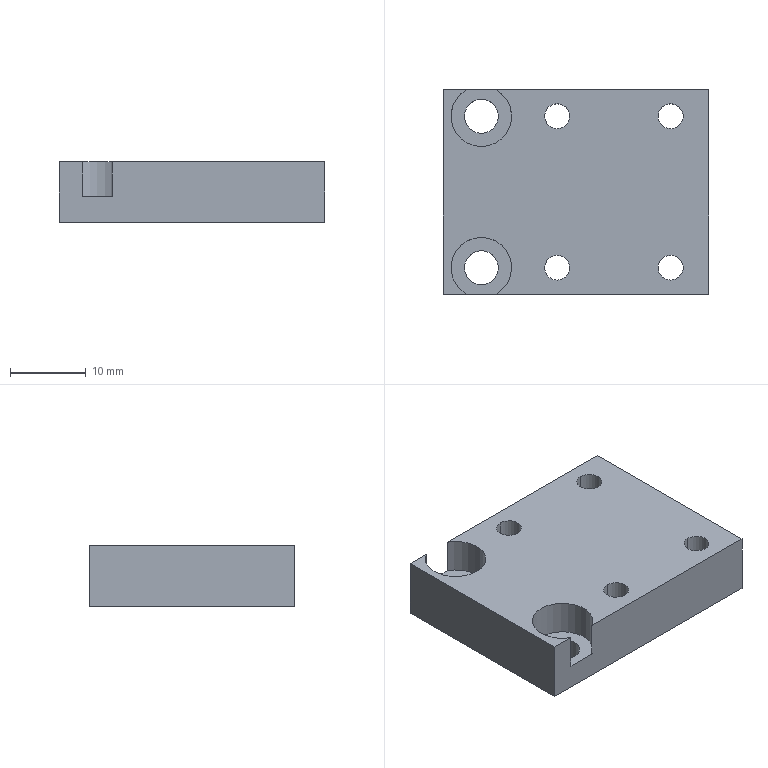Component | SolidWorks | JQ-2-0-005-1 | 1 solid | 23 faces | box 35 x 27 x 8 mm | volume 6728 mm3 | cylinder 15 | plane 8 | commonest cylinder face diameters 3.3 x8 4.5 x4 8 x3
build123d program:
from build123d import *

# Parameters (mm, degrees)
SKETCH1_W                                            = 27
SKETCH1_H                                            = 35
BOSS_EXTRUDE1_DEPTH                                  = 8
HOLE_SIZE_ACCORDING_TO_TYPE_1_OF_HEX_SOC_D           = 4.5
HOLE_SIZE_ACCORDING_TO_TYPE_1_OF_HEX_SOC_CBORE_D     = 8
HOLE_SIZE_ACCORDING_TO_TYPE_1_OF_HEX_SOC_CBORE_DEPTH = 4.6
M4_TAPPED_HOLE1_D                                    = 3.3
M4_TAPPED_HOLE1_DEPTH                                = 11.5
M4_TAPPED_HOLE1_TIP                                  = 0.9914


with BuildPart() as part:
    # Sketch1 → Boss-Extrude1 (new body)
    with BuildSketch(Plane.XY):
        with Locations((13.5, 17.5)):
            Rectangle(SKETCH1_W, SKETCH1_H)
    extrude(amount=BOSS_EXTRUDE1_DEPTH)

    # Hole Size according to type 1 of hex soc (through all)
    with Locations(Plane.XY.offset(8)):
        with Locations((23.5, 5), (3.5, 5)):
            CounterBoreHole(HOLE_SIZE_ACCORDING_TO_TYPE_1_OF_HEX_SOC_D / 2, HOLE_SIZE_ACCORDING_TO_TYPE_1_OF_HEX_SOC_CBORE_D / 2, HOLE_SIZE_ACCORDING_TO_TYPE_1_OF_HEX_SOC_CBORE_DEPTH)

    # M4 Tapped Hole1
    with Locations(Plane.XY.offset(8)):
        with Locations((23.5, 30), (3.5, 30), (3.5, 15), (23.5, 15)):
            Hole(M4_TAPPED_HOLE1_D / 2, depth=M4_TAPPED_HOLE1_DEPTH)
            with Locations((0, 0, -(M4_TAPPED_HOLE1_DEPTH + M4_TAPPED_HOLE1_TIP / 2))):  # 118° drill point
                Cone(0, M4_TAPPED_HOLE1_D / 2, M4_TAPPED_HOLE1_TIP, mode=Mode.SUBTRACT)


solid = part.part

# Placed as in the assembly
solid = solid.moved(Location((-170.058, 42.839, 99.131), (0, 0, -90)))
STEP:
#1=CARTESIAN_POINT('',(-5.514,0.6964,3.903));
#2=VERTEX_POINT('',#1);
#3=CARTESIAN_POINT('',(-5.514,0.8263,3.903));
#4=VERTEX_POINT('',#3);
#5=CARTESIAN_POINT('',(-5.514,0.7614,3.903));
#6=DIRECTION('',(-0.,-0.,-1.));
#7=DIRECTION('',(0.,1.,0.));
#8=AXIS2_PLACEMENT_3D('',#5,#6,#7);
#9=CIRCLE('',#8,0.06496);
#10=EDGE_CURVE('',#2,#4,#9,.T.);
#11=ORIENTED_EDGE('',*,*,#10,.T.);
#12=CARTESIAN_POINT('',(-5.514,0.8263,4.218));
#13=VERTEX_POINT('',#12);
#14=CARTESIAN_POINT('',(-5.514,0.8263,4.218));
#15=DIRECTION('',(0.,0.,1.));
#16=VECTOR('',#15,39.37);
#17=LINE('',#14,#16);
#18=EDGE_CURVE('',#4,#13,#17,.T.);
#19=ORIENTED_EDGE('',*,*,#18,.T.);
#20=CARTESIAN_POINT('',(-5.514,0.6964,4.218));
#21=VERTEX_POINT('',#20);
#22=CARTESIAN_POINT('',(-5.514,0.7614,4.218));
#23=DIRECTION('',(0.,0.,1.));
#24=DIRECTION('',(0.,-1.,0.));
#25=AXIS2_PLACEMENT_3D('',#22,#23,#24);
#26=CIRCLE('',#25,0.06496);
#27=EDGE_CURVE('',#13,#21,#26,.T.);
#28=ORIENTED_EDGE('',*,*,#27,.T.);
#29=CARTESIAN_POINT('',(-5.514,0.6964,4.218));
#30=DIRECTION('',(0.,0.,1.));
#31=VECTOR('',#30,39.37);
#32=LINE('',#29,#31);
#33=EDGE_CURVE('',#2,#21,#32,.T.);
#34=ORIENTED_EDGE('',*,*,#33,.F.);
#35=EDGE_LOOP('',(#11,#19,#28,#34));
#36=FACE_OUTER_BOUND('',#35,.T.);
#37=CARTESIAN_POINT('',(-5.514,0.7614,4.218));
#38=DIRECTION('',(0.,0.,1.));
#39=DIRECTION('',(0.,-1.,0.));
#40=AXIS2_PLACEMENT_3D('',#37,#38,#39);
#41=CYLINDRICAL_SURFACE('',#40,0.06496);
#42=ADVANCED_FACE('',(#36),#41,.F.);
#43=CARTESIAN_POINT('',(-5.514,1.484,3.903));
#44=VERTEX_POINT('',#43);
#45=CARTESIAN_POINT('',(-5.514,1.614,3.903));
#46=VERTEX_POINT('',#45);
#47=CARTESIAN_POINT('',(-5.514,1.549,3.903));
#48=DIRECTION('',(-0.,-0.,-1.));
#49=DIRECTION('',(0.,1.,0.));
#50=AXIS2_PLACEMENT_3D('',#47,#48,#49);
#51=CIRCLE('',#50,0.06496);
#52=EDGE_CURVE('',#44,#46,#51,.T.);
#53=ORIENTED_EDGE('',*,*,#52,.T.);
#54=CARTESIAN_POINT('',(-5.514,1.614,4.218));
#55=VERTEX_POINT('',#54);
#56=CARTESIAN_POINT('',(-5.514,1.614,4.218));
#57=DIRECTION('',(0.,0.,1.));
#58=VECTOR('',#57,39.37);
#59=LINE('',#56,#58);
#60=EDGE_CURVE('',#46,#55,#59,.T.);
#61=ORIENTED_EDGE('',*,*,#60,.T.);
#62=CARTESIAN_POINT('',(-5.514,1.484,4.218));
#63=VERTEX_POINT('',#62);
#64=CARTESIAN_POINT('',(-5.514,1.549,4.218));
#65=DIRECTION('',(0.,0.,1.));
#66=DIRECTION('',(0.,-1.,0.));
#67=AXIS2_PLACEMENT_3D('',#64,#65,#66);
#68=CIRCLE('',#67,0.06496);
#69=EDGE_CURVE('',#55,#63,#68,.T.);
#70=ORIENTED_EDGE('',*,*,#69,.T.);
#71=CARTESIAN_POINT('',(-5.514,1.484,4.218));
#72=DIRECTION('',(0.,0.,1.));
#73=VECTOR('',#72,39.37);
#74=LINE('',#71,#73);
#75=EDGE_CURVE('',#44,#63,#74,.T.);
#76=ORIENTED_EDGE('',*,*,#75,.F.);
#77=EDGE_LOOP('',(#53,#61,#70,#76));
#78=FACE_OUTER_BOUND('',#77,.T.);
#79=CARTESIAN_POINT('',(-5.514,1.549,4.218));
#80=DIRECTION('',(0.,0.,1.));
#81=DIRECTION('',(0.,-1.,0.));
#82=AXIS2_PLACEMENT_3D('',#79,#80,#81);
#83=CYLINDRICAL_SURFACE('',#82,0.06496);
#84=ADVANCED_FACE('',(#78),#83,.F.);
#85=CARTESIAN_POINT('',(-6.105,1.484,3.903));
#86=VERTEX_POINT('',#85);
#87=CARTESIAN_POINT('',(-6.105,1.614,3.903));
#88=VERTEX_POINT('',#87);
#89=CARTESIAN_POINT('',(-6.105,1.549,3.903));
#90=DIRECTION('',(-0.,-0.,-1.));
#91=DIRECTION('',(0.,1.,0.));
#92=AXIS2_PLACEMENT_3D('',#89,#90,#91);
#93=CIRCLE('',#92,0.06496);
#94=EDGE_CURVE('',#86,#88,#93,.T.);
#95=ORIENTED_EDGE('',*,*,#94,.T.);
#96=CARTESIAN_POINT('',(-6.105,1.614,4.218));
#97=VERTEX_POINT('',#96);
#98=CARTESIAN_POINT('',(-6.105,1.614,4.218));
#99=DIRECTION('',(0.,0.,1.));
#100=VECTOR('',#99,39.37);
#101=LINE('',#98,#100);
#102=EDGE_CURVE('',#88,#97,#101,.T.);
#103=ORIENTED_EDGE('',*,*,#102,.T.);
#104=CARTESIAN_POINT('',(-6.105,1.484,4.218));
#105=VERTEX_POINT('',#104);
#106=CARTESIAN_POINT('',(-6.105,1.549,4.218));
#107=DIRECTION('',(0.,0.,1.));
#108=DIRECTION('',(0.,-1.,0.));
#109=AXIS2_PLACEMENT_3D('',#106,#107,#108);
#110=CIRCLE('',#109,0.06496);
#111=EDGE_CURVE('',#97,#105,#110,.T.);
#112=ORIENTED_EDGE('',*,*,#111,.T.);
#113=CARTESIAN_POINT('',(-6.105,1.484,4.218));
#114=DIRECTION('',(0.,0.,1.));
#115=VECTOR('',#114,39.37);
#116=LINE('',#113,#115);
#117=EDGE_CURVE('',#86,#105,#116,.T.);
#118=ORIENTED_EDGE('',*,*,#117,.F.);
#119=EDGE_LOOP('',(#95,#103,#112,#118));
#120=FACE_OUTER_BOUND('',#119,.T.);
#121=CARTESIAN_POINT('',(-6.105,1.549,4.218));
#122=DIRECTION('',(0.,0.,1.));
#123=DIRECTION('',(0.,-1.,0.));
#124=AXIS2_PLACEMENT_3D('',#121,#122,#123);
#125=CYLINDRICAL_SURFACE('',#124,0.06496);
#126=ADVANCED_FACE('',(#120),#125,.F.);
#127=CARTESIAN_POINT('',(-6.105,0.6964,3.903));
#128=VERTEX_POINT('',#127);
#129=CARTESIAN_POINT('',(-6.105,0.8263,3.903));
#130=VERTEX_POINT('',#129);
#131=CARTESIAN_POINT('',(-6.105,0.7614,3.903));
#132=DIRECTION('',(-0.,-0.,-1.));
#133=DIRECTION('',(0.,1.,0.));
#134=AXIS2_PLACEMENT_3D('',#131,#132,#133);
#135=CIRCLE('',#134,0.06496);
#136=EDGE_CURVE('',#128,#130,#135,.T.);
#137=ORIENTED_EDGE('',*,*,#136,.T.);
#138=CARTESIAN_POINT('',(-6.105,0.8263,4.218));
#139=VERTEX_POINT('',#138);
#140=CARTESIAN_POINT('',(-6.105,0.8263,4.218));
#141=DIRECTION('',(0.,0.,1.));
#142=VECTOR('',#141,39.37);
#143=LINE('',#140,#142);
#144=EDGE_CURVE('',#130,#139,#143,.T.);
#145=ORIENTED_EDGE('',*,*,#144,.T.);
#146=CARTESIAN_POINT('',(-6.105,0.6964,4.218));
#147=VERTEX_POINT('',#146);
#148=CARTESIAN_POINT('',(-6.105,0.7614,4.218));
#149=DIRECTION('',(0.,0.,1.));
#150=DIRECTION('',(0.,-1.,0.));
#151=AXIS2_PLACEMENT_3D('',#148,#149,#150);
#152=CIRCLE('',#151,0.06496);
#153=EDGE_CURVE('',#139,#147,#152,.T.);
#154=ORIENTED_EDGE('',*,*,#153,.T.);
#155=CARTESIAN_POINT('',(-6.105,0.6964,4.218));
#156=DIRECTION('',(0.,0.,1.));
#157=VECTOR('',#156,39.37);
#158=LINE('',#155,#157);
#159=EDGE_CURVE('',#128,#147,#158,.T.);
#160=ORIENTED_EDGE('',*,*,#159,.F.);
#161=EDGE_LOOP('',(#137,#145,#154,#160));
#162=FACE_OUTER_BOUND('',#161,.T.);
#163=CARTESIAN_POINT('',(-6.105,0.7614,4.218));
#164=DIRECTION('',(0.,0.,1.));
#165=DIRECTION('',(0.,-1.,0.));
#166=AXIS2_PLACEMENT_3D('',#163,#164,#165);
#167=CYLINDRICAL_SURFACE('',#166,0.06496);
#168=ADVANCED_FACE('',(#162),#167,.F.);
#169=CARTESIAN_POINT('',(-6.498,0.85,3.903));
#170=VERTEX_POINT('',#169);
#171=CARTESIAN_POINT('',(-6.498,0.6728,3.903));
#172=VERTEX_POINT('',#171);
#173=CARTESIAN_POINT('',(-6.498,0.7614,3.903));
#174=DIRECTION('',(0.,0.,1.));
#175=DIRECTION('',(0.,-1.,0.));
#176=AXIS2_PLACEMENT_3D('',#173,#174,#175);
#177=CIRCLE('',#176,0.08858);
#178=EDGE_CURVE('',#170,#172,#177,.T.);
#179=ORIENTED_EDGE('',*,*,#178,.F.);
#180=CARTESIAN_POINT('',(-6.498,0.85,4.037));
#181=VERTEX_POINT('',#180);
#182=CARTESIAN_POINT('',(-6.498,0.85,4.218));
#183=DIRECTION('',(0.,0.,1.));
#184=VECTOR('',#183,39.37);
#185=LINE('',#182,#184);
#186=EDGE_CURVE('',#170,#181,#185,.T.);
#187=ORIENTED_EDGE('',*,*,#186,.T.);
#188=CARTESIAN_POINT('',(-6.498,0.6728,4.037));
#189=VERTEX_POINT('',#188);
#190=CARTESIAN_POINT('',(-6.498,0.7614,4.037));
#191=DIRECTION('',(0.,0.,1.));
#192=DIRECTION('',(0.,-1.,0.));
#193=AXIS2_PLACEMENT_3D('',#190,#191,#192);
#194=CIRCLE('',#193,0.08858);
#195=EDGE_CURVE('',#181,#189,#194,.T.);
#196=ORIENTED_EDGE('',*,*,#195,.T.);
#197=CARTESIAN_POINT('',(-6.498,0.6728,4.218));
#198=DIRECTION('',(0.,0.,1.));
#199=VECTOR('',#198,39.37);
#200=LINE('',#197,#199);
#201=EDGE_CURVE('',#172,#189,#200,.T.);
#202=ORIENTED_EDGE('',*,*,#201,.F.);
#203=EDGE_LOOP('',(#179,#187,#196,#202));
#204=FACE_OUTER_BOUND('',#203,.T.);
#205=CARTESIAN_POINT('',(-6.498,0.7614,4.218));
#206=DIRECTION('',(0.,0.,1.));
#207=DIRECTION('',(0.,-1.,0.));
#208=AXIS2_PLACEMENT_3D('',#205,#206,#207);
#209=CYLINDRICAL_SURFACE('',#208,0.08858);
#210=ADVANCED_FACE('',(#204),#209,.F.);
#211=CARTESIAN_POINT('',(-6.498,1.637,3.903));
#212=VERTEX_POINT('',#211);
#213=CARTESIAN_POINT('',(-6.498,1.46,3.903));
#214=VERTEX_POINT('',#213);
#215=CARTESIAN_POINT('',(-6.498,1.549,3.903));
#216=DIRECTION('',(0.,0.,1.));
#217=DIRECTION('',(0.,-1.,0.));
#218=AXIS2_PLACEMENT_3D('',#215,#216,#217);
#219=CIRCLE('',#218,0.08858);
#220=EDGE_CURVE('',#212,#214,#219,.T.);
#221=ORIENTED_EDGE('',*,*,#220,.F.);
#222=CARTESIAN_POINT('',(-6.498,1.637,4.037));
#223=VERTEX_POINT('',#222);
#224=CARTESIAN_POINT('',(-6.498,1.637,4.218));
#225=DIRECTION('',(0.,0.,1.));
#226=VECTOR('',#225,39.37);
#227=LINE('',#224,#226);
#228=EDGE_CURVE('',#212,#223,#227,.T.);
#229=ORIENTED_EDGE('',*,*,#228,.T.);
#230=CARTESIAN_POINT('',(-6.498,1.46,4.037));
#231=VERTEX_POINT('',#230);
#232=CARTESIAN_POINT('',(-6.498,1.549,4.037));
#233=DIRECTION('',(0.,0.,1.));
#234=DIRECTION('',(0.,-1.,0.));
#235=AXIS2_PLACEMENT_3D('',#232,#233,#234);
#236=CIRCLE('',#235,0.08858);
#237=EDGE_CURVE('',#223,#231,#236,.T.);
#238=ORIENTED_EDGE('',*,*,#237,.T.);
#239=CARTESIAN_POINT('',(-6.498,1.46,4.218));
#240=DIRECTION('',(0.,0.,1.));
#241=VECTOR('',#240,39.37);
#242=LINE('',#239,#241);
#243=EDGE_CURVE('',#214,#231,#242,.T.);
#244=ORIENTED_EDGE('',*,*,#243,.F.);
#245=EDGE_LOOP('',(#221,#229,#238,#244));
#246=FACE_OUTER_BOUND('',#245,.T.);
#247=CARTESIAN_POINT('',(-6.498,1.549,4.218));
#248=DIRECTION('',(0.,0.,1.));
#249=DIRECTION('',(0.,-1.,0.));
#250=AXIS2_PLACEMENT_3D('',#247,#248,#249);
#251=CYLINDRICAL_SURFACE('',#250,0.08858);
#252=ADVANCED_FACE('',(#246),#251,.F.);
#253=CARTESIAN_POINT('',(-6.498,1.391,4.037));
#254=VERTEX_POINT('',#253);
#255=CARTESIAN_POINT('',(-6.422,1.687,4.037));
#256=VERTEX_POINT('',#255);
#257=CARTESIAN_POINT('',(-6.498,1.549,4.037));
#258=DIRECTION('',(0.,0.,1.));
#259=DIRECTION('',(0.,-1.,0.));
#260=AXIS2_PLACEMENT_3D('',#257,#258,#259);
#261=CIRCLE('',#260,0.1575);
#262=EDGE_CURVE('',#254,#256,#261,.T.);
#263=ORIENTED_EDGE('',*,*,#262,.F.);
#264=CARTESIAN_POINT('',(-6.498,1.391,4.218));
#265=VERTEX_POINT('',#264);
#266=CARTESIAN_POINT('',(-6.498,1.391,4.218));
#267=DIRECTION('',(0.,0.,1.));
#268=VECTOR('',#267,39.37);
#269=LINE('',#266,#268);
#270=EDGE_CURVE('',#254,#265,#269,.T.);
#271=ORIENTED_EDGE('',*,*,#270,.T.);
#272=CARTESIAN_POINT('',(-6.422,1.687,4.218));
#273=VERTEX_POINT('',#272);
#274=CARTESIAN_POINT('',(-6.498,1.549,4.218));
#275=DIRECTION('',(-0.,-0.,-1.));
#276=DIRECTION('',(0.,1.,0.));
#277=AXIS2_PLACEMENT_3D('',#274,#275,#276);
#278=CIRCLE('',#277,0.1575);
#279=EDGE_CURVE('',#273,#265,#278,.T.);
#280=ORIENTED_EDGE('',*,*,#279,.F.);
#281=CARTESIAN_POINT('',(-6.422,1.687,4.218));
#282=DIRECTION('',(0.,0.,1.));
#283=VECTOR('',#282,39.37);
#284=LINE('',#281,#283);
#285=EDGE_CURVE('',#256,#273,#284,.T.);
#286=ORIENTED_EDGE('',*,*,#285,.F.);
#287=EDGE_LOOP('',(#263,#271,#280,#286));
#288=FACE_OUTER_BOUND('',#287,.T.);
#289=CARTESIAN_POINT('',(-6.498,1.549,4.218));
#290=DIRECTION('',(0.,0.,1.));
#291=DIRECTION('',(0.,-1.,0.));
#292=AXIS2_PLACEMENT_3D('',#289,#290,#291);
#293=CYLINDRICAL_SURFACE('',#292,0.1575);
#294=ADVANCED_FACE('',(#288),#293,.F.);
#295=CARTESIAN_POINT('',(-6.575,1.687,4.037));
#296=VERTEX_POINT('',#295);
#297=CARTESIAN_POINT('',(-6.695,1.687,4.037));
#298=DIRECTION('',(1.,-0.,-0.));
#299=VECTOR('',#298,39.37);
#300=LINE('',#297,#299);
#301=EDGE_CURVE('',#296,#256,#300,.T.);
#302=ORIENTED_EDGE('',*,*,#301,.T.);
#303=ORIENTED_EDGE('',*,*,#285,.T.);
#304=CARTESIAN_POINT('',(-5.317,1.687,4.218));
#305=VERTEX_POINT('',#304);
#306=CARTESIAN_POINT('',(-6.695,1.687,4.218));
#307=DIRECTION('',(-1.,0.,0.));
#308=VECTOR('',#307,39.37);
#309=LINE('',#306,#308);
#310=EDGE_CURVE('',#305,#273,#309,.T.);
#311=ORIENTED_EDGE('',*,*,#310,.F.);
#312=CARTESIAN_POINT('',(-5.317,1.687,3.903));
#313=VERTEX_POINT('',#312);
#314=CARTESIAN_POINT('',(-5.317,1.687,4.218));
#315=DIRECTION('',(-0.,-0.,-1.));
#316=VECTOR('',#315,39.37);
#317=LINE('',#314,#316);
#318=EDGE_CURVE('',#305,#313,#317,.T.);
#319=ORIENTED_EDGE('',*,*,#318,.T.);
#320=CARTESIAN_POINT('',(-6.695,1.687,3.903));
#321=VERTEX_POINT('',#320);
#322=CARTESIAN_POINT('',(-6.695,1.687,3.903));
#323=DIRECTION('',(-1.,0.,0.));
#324=VECTOR('',#323,39.37);
#325=LINE('',#322,#324);
#326=EDGE_CURVE('',#313,#321,#325,.T.);
#327=ORIENTED_EDGE('',*,*,#326,.T.);
#328=CARTESIAN_POINT('',(-6.695,1.687,4.218));
#329=VERTEX_POINT('',#328);
#330=CARTESIAN_POINT('',(-6.695,1.687,4.218));
#331=DIRECTION('',(-0.,-0.,-1.));
#332=VECTOR('',#331,39.37);
#333=LINE('',#330,#332);
#334=EDGE_CURVE('',#329,#321,#333,.T.);
#335=ORIENTED_EDGE('',*,*,#334,.F.);
#336=CARTESIAN_POINT('',(-6.575,1.687,4.218));
#337=VERTEX_POINT('',#336);
#338=CARTESIAN_POINT('',(-6.695,1.687,4.218));
#339=DIRECTION('',(-1.,0.,0.));
#340=VECTOR('',#339,39.37);
#341=LINE('',#338,#340);
#342=EDGE_CURVE('',#337,#329,#341,.T.);
#343=ORIENTED_EDGE('',*,*,#342,.F.);
#344=CARTESIAN_POINT('',(-6.575,1.687,4.218));
#345=DIRECTION('',(-0.,-0.,-1.));
#346=VECTOR('',#345,39.37);
#347=LINE('',#344,#346);
#348=EDGE_CURVE('',#337,#296,#347,.T.);
#349=ORIENTED_EDGE('',*,*,#348,.T.);
#350=EDGE_LOOP('',(#302,#303,#311,#319,#327,#335,#343,#349));
#351=FACE_OUTER_BOUND('',#350,.T.);
#352=CARTESIAN_POINT('',(-6.695,1.687,4.218));
#353=DIRECTION('',(-0.,-1.,0.));
#354=DIRECTION('',(-0.,-0.,-1.));
#355=AXIS2_PLACEMENT_3D('',#352,#353,#354);
#356=PLANE('',#355);
#357=ADVANCED_FACE('',(#351),#356,.F.);
#358=CARTESIAN_POINT('',(-6.695,0.6236,3.903));
#359=VERTEX_POINT('',#358);
#360=CARTESIAN_POINT('',(-6.695,1.687,3.903));
#361=DIRECTION('',(-0.,-1.,0.));
#362=VECTOR('',#361,39.37);
#363=LINE('',#360,#362);
#364=EDGE_CURVE('',#321,#359,#363,.T.);
#365=ORIENTED_EDGE('',*,*,#364,.T.);
#366=CARTESIAN_POINT('',(-6.695,0.6236,4.218));
#367=VERTEX_POINT('',#366);
#368=CARTESIAN_POINT('',(-6.695,0.6236,4.218));
#369=DIRECTION('',(-0.,-0.,-1.));
#370=VECTOR('',#369,39.37);
#371=LINE('',#368,#370);
#372=EDGE_CURVE('',#367,#359,#371,.T.);
#373=ORIENTED_EDGE('',*,*,#372,.F.);
#374=CARTESIAN_POINT('',(-6.695,1.687,4.218));
#375=DIRECTION('',(-0.,-1.,0.));
#376=VECTOR('',#375,39.37);
#377=LINE('',#374,#376);
#378=EDGE_CURVE('',#329,#367,#377,.T.);
#379=ORIENTED_EDGE('',*,*,#378,.F.);
#380=ORIENTED_EDGE('',*,*,#334,.T.);
#381=EDGE_LOOP('',(#365,#373,#379,#380));
#382=FACE_OUTER_BOUND('',#381,.T.);
#383=CARTESIAN_POINT('',(-6.695,1.687,4.218));
#384=DIRECTION('',(1.,-0.,-0.));
#385=DIRECTION('',(0.,0.,1.));
#386=AXIS2_PLACEMENT_3D('',#383,#384,#385);
#387=PLANE('',#386);
#388=ADVANCED_FACE('',(#382),#387,.F.);
#389=CARTESIAN_POINT('',(-6.422,0.6236,4.037));
#390=VERTEX_POINT('',#389);
#391=CARTESIAN_POINT('',(-6.575,0.6236,4.037));
#392=VERTEX_POINT('',#391);
#393=CARTESIAN_POINT('',(-6.695,0.6236,4.037));
#394=DIRECTION('',(-1.,0.,0.));
#395=VECTOR('',#394,39.37);
#396=LINE('',#393,#395);
#397=EDGE_CURVE('',#390,#392,#396,.T.);
#398=ORIENTED_EDGE('',*,*,#397,.T.);
#399=CARTESIAN_POINT('',(-6.575,0.6236,4.218));
#400=VERTEX_POINT('',#399);
#401=CARTESIAN_POINT('',(-6.575,0.6236,4.218));
#402=DIRECTION('',(0.,0.,1.));
#403=VECTOR('',#402,39.37);
#404=LINE('',#401,#403);
#405=EDGE_CURVE('',#392,#400,#404,.T.);
#406=ORIENTED_EDGE('',*,*,#405,.T.);
#407=CARTESIAN_POINT('',(-6.695,0.6236,4.218));
#408=DIRECTION('',(1.,-0.,-0.));
#409=VECTOR('',#408,39.37);
#410=LINE('',#407,#409);
#411=EDGE_CURVE('',#367,#400,#410,.T.);
#412=ORIENTED_EDGE('',*,*,#411,.F.);
#413=ORIENTED_EDGE('',*,*,#372,.T.);
#414=CARTESIAN_POINT('',(-5.317,0.6236,3.903));
#415=VERTEX_POINT('',#414);
#416=CARTESIAN_POINT('',(-6.695,0.6236,3.903));
#417=DIRECTION('',(1.,-0.,-0.));
#418=VECTOR('',#417,39.37);
#419=LINE('',#416,#418);
#420=EDGE_CURVE('',#359,#415,#419,.T.);
#421=ORIENTED_EDGE('',*,*,#420,.T.);
#422=CARTESIAN_POINT('',(-5.317,0.6236,4.218));
#423=VERTEX_POINT('',#422);
#424=CARTESIAN_POINT('',(-5.317,0.6236,4.218));
#425=DIRECTION('',(-0.,-0.,-1.));
#426=VECTOR('',#425,39.37);
#427=LINE('',#424,#426);
#428=EDGE_CURVE('',#423,#415,#427,.T.);
#429=ORIENTED_EDGE('',*,*,#428,.F.);
#430=CARTESIAN_POINT('',(-6.422,0.6236,4.218));
#431=VERTEX_POINT('',#430);
#432=CARTESIAN_POINT('',(-6.695,0.6236,4.218));
#433=DIRECTION('',(1.,-0.,-0.));
#434=VECTOR('',#433,39.37);
#435=LINE('',#432,#434);
#436=EDGE_CURVE('',#431,#423,#435,.T.);
#437=ORIENTED_EDGE('',*,*,#436,.F.);
#438=CARTESIAN_POINT('',(-6.422,0.6236,4.218));
#439=DIRECTION('',(-0.,-0.,-1.));
#440=VECTOR('',#439,39.37);
#441=LINE('',#438,#440);
#442=EDGE_CURVE('',#431,#390,#441,.T.);
#443=ORIENTED_EDGE('',*,*,#442,.T.);
#444=EDGE_LOOP('',(#398,#406,#412,#413,#421,#429,#437,#443));
#445=FACE_OUTER_BOUND('',#444,.T.);
#446=CARTESIAN_POINT('',(-6.695,0.6236,4.218));
#447=DIRECTION('',(0.,1.,-0.));
#448=DIRECTION('',(0.,0.,1.));
#449=AXIS2_PLACEMENT_3D('',#446,#447,#448);
#450=PLANE('',#449);
#451=ADVANCED_FACE('',(#445),#450,.F.);
#452=CARTESIAN_POINT('',(-5.317,1.687,3.903));
#453=DIRECTION('',(0.,1.,-0.));
#454=VECTOR('',#453,39.37);
#455=LINE('',#452,#454);
#456=EDGE_CURVE('',#415,#313,#455,.T.);
#457=ORIENTED_EDGE('',*,*,#456,.T.);
#458=ORIENTED_EDGE('',*,*,#318,.F.);
#459=CARTESIAN_POINT('',(-5.317,1.687,4.218));
#460=DIRECTION('',(0.,1.,-0.));
#461=VECTOR('',#460,39.37);
#462=LINE('',#459,#461);
#463=EDGE_CURVE('',#423,#305,#462,.T.);
#464=ORIENTED_EDGE('',*,*,#463,.F.);
#465=ORIENTED_EDGE('',*,*,#428,.T.);
#466=EDGE_LOOP('',(#457,#458,#464,#465));
#467=FACE_OUTER_BOUND('',#466,.T.);
#468=CARTESIAN_POINT('',(-5.317,1.687,4.218));
#469=DIRECTION('',(-1.,0.,0.));
#470=DIRECTION('',(-0.,-0.,-1.));
#471=AXIS2_PLACEMENT_3D('',#468,#469,#470);
#472=PLANE('',#471);
#473=ADVANCED_FACE('',(#467),#472,.F.);
#474=CARTESIAN_POINT('',(-5.514,0.7614,4.218));
#475=DIRECTION('',(0.,0.,1.));
#476=DIRECTION('',(0.,-1.,0.));
#477=AXIS2_PLACEMENT_3D('',#474,#475,#476);
#478=CIRCLE('',#477,0.06496);
#479=EDGE_CURVE('',#21,#13,#478,.T.);
#480=ORIENTED_EDGE('',*,*,#479,.F.);
#481=ORIENTED_EDGE('',*,*,#27,.F.);
#482=EDGE_LOOP('',(#480,#481));
#483=FACE_BOUND('',#482,.T.);
#484=CARTESIAN_POINT('',(-5.514,1.549,4.218));
#485=DIRECTION('',(0.,0.,1.));
#486=DIRECTION('',(0.,-1.,0.));
#487=AXIS2_PLACEMENT_3D('',#484,#485,#486);
#488=CIRCLE('',#487,0.06496);
#489=EDGE_CURVE('',#63,#55,#488,.T.);
#490=ORIENTED_EDGE('',*,*,#489,.F.);
#491=ORIENTED_EDGE('',*,*,#69,.F.);
#492=EDGE_LOOP('',(#490,#491));
#493=FACE_BOUND('',#492,.T.);
#494=CARTESIAN_POINT('',(-6.105,1.549,4.218));
#495=DIRECTION('',(0.,0.,1.));
#496=DIRECTION('',(0.,-1.,0.));
#497=AXIS2_PLACEMENT_3D('',#494,#495,#496);
#498=CIRCLE('',#497,0.06496);
#499=EDGE_CURVE('',#105,#97,#498,.T.);
#500=ORIENTED_EDGE('',*,*,#499,.F.);
#501=ORIENTED_EDGE('',*,*,#111,.F.);
#502=EDGE_LOOP('',(#500,#501));
#503=FACE_BOUND('',#502,.T.);
#504=CARTESIAN_POINT('',(-6.105,0.7614,4.218));
#505=DIRECTION('',(0.,0.,1.));
#506=DIRECTION('',(0.,-1.,0.));
#507=AXIS2_PLACEMENT_3D('',#504,#505,#506);
#508=CIRCLE('',#507,0.06496);
#509=EDGE_CURVE('',#147,#139,#508,.T.);
#510=ORIENTED_EDGE('',*,*,#509,.F.);
#511=ORIENTED_EDGE('',*,*,#153,.F.);
#512=EDGE_LOOP('',(#510,#511));
#513=FACE_BOUND('',#512,.T.);
#514=ORIENTED_EDGE('',*,*,#411,.T.);
#515=CARTESIAN_POINT('',(-6.498,0.7614,4.218));
#516=DIRECTION('',(0.,0.,1.));
#517=DIRECTION('',(0.,-1.,0.));
#518=AXIS2_PLACEMENT_3D('',#515,#516,#517);
#519=CIRCLE('',#518,0.1575);
#520=EDGE_CURVE('',#431,#400,#519,.T.);
#521=ORIENTED_EDGE('',*,*,#520,.F.);
#522=ORIENTED_EDGE('',*,*,#436,.T.);
#523=ORIENTED_EDGE('',*,*,#463,.T.);
#524=ORIENTED_EDGE('',*,*,#310,.T.);
#525=ORIENTED_EDGE('',*,*,#279,.T.);
#526=CARTESIAN_POINT('',(-6.498,1.549,4.218));
#527=DIRECTION('',(-0.,-0.,-1.));
#528=DIRECTION('',(0.,1.,0.));
#529=AXIS2_PLACEMENT_3D('',#526,#527,#528);
#530=CIRCLE('',#529,0.1575);
#531=EDGE_CURVE('',#265,#337,#530,.T.);
#532=ORIENTED_EDGE('',*,*,#531,.T.);
#533=ORIENTED_EDGE('',*,*,#342,.T.);
#534=ORIENTED_EDGE('',*,*,#378,.T.);
#535=EDGE_LOOP('',(#514,#521,#522,#523,#524,#525,#532,#533,#534));
#536=FACE_OUTER_BOUND('',#535,.T.);
#537=CARTESIAN_POINT('',(-5.317,1.687,4.218));
#538=DIRECTION('',(-0.,-0.,-1.));
#539=DIRECTION('',(0.,1.,-0.));
#540=AXIS2_PLACEMENT_3D('',#537,#538,#539);
#541=PLANE('',#540);
#542=ADVANCED_FACE('',(#483,#493,#503,#513,#536),#541,.F.);
#543=ORIENTED_EDGE('',*,*,#10,.F.);
#544=CARTESIAN_POINT('',(-5.514,0.7614,3.903));
#545=DIRECTION('',(-0.,-0.,-1.));
#546=DIRECTION('',(0.,1.,0.));
#547=AXIS2_PLACEMENT_3D('',#544,#545,#546);
#548=CIRCLE('',#547,0.06496);
#549=EDGE_CURVE('',#4,#2,#548,.T.);
#550=ORIENTED_EDGE('',*,*,#549,.F.);
#551=EDGE_LOOP('',(#543,#550));
#552=FACE_BOUND('',#551,.T.);
#553=ORIENTED_EDGE('',*,*,#52,.F.);
#554=CARTESIAN_POINT('',(-5.514,1.549,3.903));
#555=DIRECTION('',(-0.,-0.,-1.));
#556=DIRECTION('',(0.,1.,0.));
#557=AXIS2_PLACEMENT_3D('',#554,#555,#556);
#558=CIRCLE('',#557,0.06496);
#559=EDGE_CURVE('',#46,#44,#558,.T.);
#560=ORIENTED_EDGE('',*,*,#559,.F.);
#561=EDGE_LOOP('',(#553,#560));
#562=FACE_BOUND('',#561,.T.);
#563=ORIENTED_EDGE('',*,*,#94,.F.);
#564=CARTESIAN_POINT('',(-6.105,1.549,3.903));
#565=DIRECTION('',(-0.,-0.,-1.));
#566=DIRECTION('',(0.,1.,0.));
#567=AXIS2_PLACEMENT_3D('',#564,#565,#566);
#568=CIRCLE('',#567,0.06496);
#569=EDGE_CURVE('',#88,#86,#568,.T.);
#570=ORIENTED_EDGE('',*,*,#569,.F.);
#571=EDGE_LOOP('',(#563,#570));
#572=FACE_BOUND('',#571,.T.);
#573=ORIENTED_EDGE('',*,*,#136,.F.);
#574=CARTESIAN_POINT('',(-6.105,0.7614,3.903));
#575=DIRECTION('',(-0.,-0.,-1.));
#576=DIRECTION('',(0.,1.,0.));
#577=AXIS2_PLACEMENT_3D('',#574,#575,#576);
#578=CIRCLE('',#577,0.06496);
#579=EDGE_CURVE('',#130,#128,#578,.T.);
#580=ORIENTED_EDGE('',*,*,#579,.F.);
#581=EDGE_LOOP('',(#573,#580));
#582=FACE_BOUND('',#581,.T.);
#583=CARTESIAN_POINT('',(-6.498,0.7614,3.903));
#584=DIRECTION('',(0.,0.,1.));
#585=DIRECTION('',(0.,-1.,0.));
#586=AXIS2_PLACEMENT_3D('',#583,#584,#585);
#587=CIRCLE('',#586,0.08858);
#588=EDGE_CURVE('',#172,#170,#587,.T.);
#589=ORIENTED_EDGE('',*,*,#588,.T.);
#590=ORIENTED_EDGE('',*,*,#178,.T.);
#591=EDGE_LOOP('',(#589,#590));
#592=FACE_BOUND('',#591,.T.);
#593=CARTESIAN_POINT('',(-6.498,1.549,3.903));
#594=DIRECTION('',(0.,0.,1.));
#595=DIRECTION('',(0.,-1.,0.));
#596=AXIS2_PLACEMENT_3D('',#593,#594,#595);
#597=CIRCLE('',#596,0.08858);
#598=EDGE_CURVE('',#214,#212,#597,.T.);
#599=ORIENTED_EDGE('',*,*,#598,.T.);
#600=ORIENTED_EDGE('',*,*,#220,.T.);
#601=EDGE_LOOP('',(#599,#600));
#602=FACE_BOUND('',#601,.T.);
#603=ORIENTED_EDGE('',*,*,#326,.F.);
#604=ORIENTED_EDGE('',*,*,#456,.F.);
#605=ORIENTED_EDGE('',*,*,#420,.F.);
#606=ORIENTED_EDGE('',*,*,#364,.F.);
#607=EDGE_LOOP('',(#603,#604,#605,#606));
#608=FACE_OUTER_BOUND('',#607,.T.);
#609=CARTESIAN_POINT('',(-5.317,1.687,3.903));
#610=DIRECTION('',(-0.,-0.,-1.));
#611=DIRECTION('',(0.,1.,-0.));
#612=AXIS2_PLACEMENT_3D('',#609,#610,#611);
#613=PLANE('',#612);
#614=ADVANCED_FACE('',(#552,#562,#572,#582,#592,#602,#608),#613,.T.);
#615=CARTESIAN_POINT('',(-6.498,1.549,4.037));
#616=DIRECTION('',(0.,0.,1.));
#617=DIRECTION('',(0.,-1.,0.));
#618=AXIS2_PLACEMENT_3D('',#615,#616,#617);
#619=CIRCLE('',#618,0.08858);
#620=EDGE_CURVE('',#231,#223,#619,.T.);
#621=ORIENTED_EDGE('',*,*,#620,.F.);
#622=ORIENTED_EDGE('',*,*,#237,.F.);
#623=EDGE_LOOP('',(#621,#622));
#624=FACE_BOUND('',#623,.T.);
#625=CARTESIAN_POINT('',(-6.498,1.549,4.037));
#626=DIRECTION('',(0.,0.,1.));
#627=DIRECTION('',(0.,-1.,0.));
#628=AXIS2_PLACEMENT_3D('',#625,#626,#627);
#629=CIRCLE('',#628,0.1575);
#630=EDGE_CURVE('',#296,#254,#629,.T.);
#631=ORIENTED_EDGE('',*,*,#630,.T.);
#632=ORIENTED_EDGE('',*,*,#262,.T.);
#633=ORIENTED_EDGE('',*,*,#301,.F.);
#634=EDGE_LOOP('',(#631,#632,#633));
#635=FACE_OUTER_BOUND('',#634,.T.);
#636=CARTESIAN_POINT('',(-6.498,1.46,4.037));
#637=DIRECTION('',(-0.,-0.,-1.));
#638=DIRECTION('',(0.,1.,-0.));
#639=AXIS2_PLACEMENT_3D('',#636,#637,#638);
#640=PLANE('',#639);
#641=ADVANCED_FACE('',(#624,#635),#640,.F.);
#642=ORIENTED_EDGE('',*,*,#270,.F.);
#643=ORIENTED_EDGE('',*,*,#630,.F.);
#644=ORIENTED_EDGE('',*,*,#348,.F.);
#645=ORIENTED_EDGE('',*,*,#531,.F.);
#646=EDGE_LOOP('',(#642,#643,#644,#645));
#647=FACE_OUTER_BOUND('',#646,.T.);
#648=CARTESIAN_POINT('',(-6.498,1.549,4.218));
#649=DIRECTION('',(0.,0.,1.));
#650=DIRECTION('',(0.,-1.,0.));
#651=AXIS2_PLACEMENT_3D('',#648,#649,#650);
#652=CYLINDRICAL_SURFACE('',#651,0.1575);
#653=ADVANCED_FACE('',(#647),#652,.F.);
#654=ORIENTED_EDGE('',*,*,#228,.F.);
#655=ORIENTED_EDGE('',*,*,#598,.F.);
#656=ORIENTED_EDGE('',*,*,#243,.T.);
#657=ORIENTED_EDGE('',*,*,#620,.T.);
#658=EDGE_LOOP('',(#654,#655,#656,#657));
#659=FACE_OUTER_BOUND('',#658,.T.);
#660=CARTESIAN_POINT('',(-6.498,1.549,4.218));
#661=DIRECTION('',(0.,0.,1.));
#662=DIRECTION('',(0.,-1.,0.));
#663=AXIS2_PLACEMENT_3D('',#660,#661,#662);
#664=CYLINDRICAL_SURFACE('',#663,0.08858);
#665=ADVANCED_FACE('',(#659),#664,.F.);
#666=CARTESIAN_POINT('',(-6.498,0.7614,4.037));
#667=DIRECTION('',(0.,0.,1.));
#668=DIRECTION('',(0.,-1.,0.));
#669=AXIS2_PLACEMENT_3D('',#666,#667,#668);
#670=CIRCLE('',#669,0.08858);
#671=EDGE_CURVE('',#189,#181,#670,.T.);
#672=ORIENTED_EDGE('',*,*,#671,.F.);
#673=ORIENTED_EDGE('',*,*,#195,.F.);
#674=EDGE_LOOP('',(#672,#673));
#675=FACE_BOUND('',#674,.T.);
#676=CARTESIAN_POINT('',(-6.498,0.7614,4.037));
#677=DIRECTION('',(0.,0.,1.));
#678=DIRECTION('',(0.,-1.,0.));
#679=AXIS2_PLACEMENT_3D('',#676,#677,#678);
#680=CIRCLE('',#679,0.1575);
#681=EDGE_CURVE('',#390,#392,#680,.T.);
#682=ORIENTED_EDGE('',*,*,#681,.T.);
#683=ORIENTED_EDGE('',*,*,#397,.F.);
#684=EDGE_LOOP('',(#682,#683));
#685=FACE_OUTER_BOUND('',#684,.T.);
#686=CARTESIAN_POINT('',(-6.498,0.6728,4.037));
#687=DIRECTION('',(-0.,-0.,-1.));
#688=DIRECTION('',(0.,1.,-0.));
#689=AXIS2_PLACEMENT_3D('',#686,#687,#688);
#690=PLANE('',#689);
#691=ADVANCED_FACE('',(#675,#685),#690,.F.);
#692=ORIENTED_EDGE('',*,*,#681,.F.);
#693=ORIENTED_EDGE('',*,*,#442,.F.);
#694=ORIENTED_EDGE('',*,*,#520,.T.);
#695=ORIENTED_EDGE('',*,*,#405,.F.);
#696=EDGE_LOOP('',(#692,#693,#694,#695));
#697=FACE_OUTER_BOUND('',#696,.T.);
#698=CARTESIAN_POINT('',(-6.498,0.7614,4.218));
#699=DIRECTION('',(0.,0.,1.));
#700=DIRECTION('',(0.,-1.,0.));
#701=AXIS2_PLACEMENT_3D('',#698,#699,#700);
#702=CYLINDRICAL_SURFACE('',#701,0.1575);
#703=ADVANCED_FACE('',(#697),#702,.F.);
#704=ORIENTED_EDGE('',*,*,#186,.F.);
#705=ORIENTED_EDGE('',*,*,#588,.F.);
#706=ORIENTED_EDGE('',*,*,#201,.T.);
#707=ORIENTED_EDGE('',*,*,#671,.T.);
#708=EDGE_LOOP('',(#704,#705,#706,#707));
#709=FACE_OUTER_BOUND('',#708,.T.);
#710=CARTESIAN_POINT('',(-6.498,0.7614,4.218));
#711=DIRECTION('',(0.,0.,1.));
#712=DIRECTION('',(0.,-1.,0.));
#713=AXIS2_PLACEMENT_3D('',#710,#711,#712);
#714=CYLINDRICAL_SURFACE('',#713,0.08858);
#715=ADVANCED_FACE('',(#709),#714,.F.);
#716=ORIENTED_EDGE('',*,*,#144,.F.);
#717=ORIENTED_EDGE('',*,*,#579,.T.);
#718=ORIENTED_EDGE('',*,*,#159,.T.);
#719=ORIENTED_EDGE('',*,*,#509,.T.);
#720=EDGE_LOOP('',(#716,#717,#718,#719));
#721=FACE_OUTER_BOUND('',#720,.T.);
#722=CARTESIAN_POINT('',(-6.105,0.7614,4.218));
#723=DIRECTION('',(0.,0.,1.));
#724=DIRECTION('',(0.,-1.,0.));
#725=AXIS2_PLACEMENT_3D('',#722,#723,#724);
#726=CYLINDRICAL_SURFACE('',#725,0.06496);
#727=ADVANCED_FACE('',(#721),#726,.F.);
#728=ORIENTED_EDGE('',*,*,#102,.F.);
#729=ORIENTED_EDGE('',*,*,#569,.T.);
#730=ORIENTED_EDGE('',*,*,#117,.T.);
#731=ORIENTED_EDGE('',*,*,#499,.T.);
#732=EDGE_LOOP('',(#728,#729,#730,#731));
#733=FACE_OUTER_BOUND('',#732,.T.);
#734=CARTESIAN_POINT('',(-6.105,1.549,4.218));
#735=DIRECTION('',(0.,0.,1.));
#736=DIRECTION('',(0.,-1.,0.));
#737=AXIS2_PLACEMENT_3D('',#734,#735,#736);
#738=CYLINDRICAL_SURFACE('',#737,0.06496);
#739=ADVANCED_FACE('',(#733),#738,.F.);
#740=ORIENTED_EDGE('',*,*,#60,.F.);
#741=ORIENTED_EDGE('',*,*,#559,.T.);
#742=ORIENTED_EDGE('',*,*,#75,.T.);
#743=ORIENTED_EDGE('',*,*,#489,.T.);
#744=EDGE_LOOP('',(#740,#741,#742,#743));
#745=FACE_OUTER_BOUND('',#744,.T.);
#746=CARTESIAN_POINT('',(-5.514,1.549,4.218));
#747=DIRECTION('',(0.,0.,1.));
#748=DIRECTION('',(0.,-1.,0.));
#749=AXIS2_PLACEMENT_3D('',#746,#747,#748);
#750=CYLINDRICAL_SURFACE('',#749,0.06496);
#751=ADVANCED_FACE('',(#745),#750,.F.);
#752=ORIENTED_EDGE('',*,*,#18,.F.);
#753=ORIENTED_EDGE('',*,*,#549,.T.);
#754=ORIENTED_EDGE('',*,*,#33,.T.);
#755=ORIENTED_EDGE('',*,*,#479,.T.);
#756=EDGE_LOOP('',(#752,#753,#754,#755));
#757=FACE_OUTER_BOUND('',#756,.T.);
#758=CARTESIAN_POINT('',(-5.514,0.7614,4.218));
#759=DIRECTION('',(0.,0.,1.));
#760=DIRECTION('',(0.,-1.,0.));
#761=AXIS2_PLACEMENT_3D('',#758,#759,#760);
#762=CYLINDRICAL_SURFACE('',#761,0.06496);
#763=ADVANCED_FACE('',(#757),#762,.F.);
#764=CLOSED_SHELL('',(#42,#84,#126,#168,#210,#252,#294,#357,#388,#451,#473,#542,#614,#641,#653,#665,#691,#703,#715,#727,#739,#751,#763));
#765=MANIFOLD_SOLID_BREP('',#764);
#766=CARTESIAN_POINT('',(0.,0.,0.));
#767=DIRECTION('',(0.,0.,1.));
#768=DIRECTION('',(1.,0.,0.));
#769=AXIS2_PLACEMENT_3D('',#766,#767,#768);
#770=(LENGTH_UNIT()NAMED_UNIT(*)SI_UNIT($,.METRE.));
#771=LENGTH_MEASURE_WITH_UNIT(LENGTH_MEASURE(0.0254),#770);
#772=DIMENSIONAL_EXPONENTS(1.,0.,0.,0.,0.,0.,0.);
#773=(CONVERSION_BASED_UNIT('',#771)LENGTH_UNIT()NAMED_UNIT(#772));
#774=UNCERTAINTY_MEASURE_WITH_UNIT(LENGTH_MEASURE(0.00001),#773,'','');
#775=(NAMED_UNIT(*)PLANE_ANGLE_UNIT()SI_UNIT($,.RADIAN.));
#776=(NAMED_UNIT(*)SI_UNIT($,.STERADIAN.)SOLID_ANGLE_UNIT());
#777=(GEOMETRIC_REPRESENTATION_CONTEXT(3)GLOBAL_UNCERTAINTY_ASSIGNED_CONTEXT((#774))GLOBAL_UNIT_ASSIGNED_CONTEXT((#773,#775,#776))REPRESENTATION_CONTEXT('',''));
#778=ADVANCED_BREP_SHAPE_REPRESENTATION('',(#765,#769),#777);
#779=COLOUR_RGB('',0.7922,0.8196,0.9333);
#780=FILL_AREA_STYLE_COLOUR('',#779);
#781=FILL_AREA_STYLE('',(#780));
#782=SURFACE_STYLE_FILL_AREA(#781);
#783=SURFACE_SIDE_STYLE('',(#782));
#784=SURFACE_STYLE_USAGE(.BOTH.,#783);
#785=PRESENTATION_STYLE_ASSIGNMENT((#784));
#786=STYLED_ITEM('',(#785),#765);
#787=(LENGTH_UNIT()NAMED_UNIT(*)SI_UNIT($,.METRE.));
#788=LENGTH_MEASURE_WITH_UNIT(LENGTH_MEASURE(0.0254),#787);
#789=DIMENSIONAL_EXPONENTS(1.,0.,0.,0.,0.,0.,0.);
#790=(CONVERSION_BASED_UNIT('',#788)LENGTH_UNIT()NAMED_UNIT(#789));
#791=UNCERTAINTY_MEASURE_WITH_UNIT(LENGTH_MEASURE(0.00001),#790,'','');
#792=(NAMED_UNIT(*)PLANE_ANGLE_UNIT()SI_UNIT($,.RADIAN.));
#793=(NAMED_UNIT(*)SI_UNIT($,.STERADIAN.)SOLID_ANGLE_UNIT());
#794=(GEOMETRIC_REPRESENTATION_CONTEXT(3)GLOBAL_UNCERTAINTY_ASSIGNED_CONTEXT((#791))GLOBAL_UNIT_ASSIGNED_CONTEXT((#790,#792,#793))REPRESENTATION_CONTEXT('',''));
#795=MECHANICAL_DESIGN_GEOMETRIC_PRESENTATION_REPRESENTATION('',(#786),#794);
#796=PRESENTATION_LAYER_ASSIGNMENT('','',(#786));